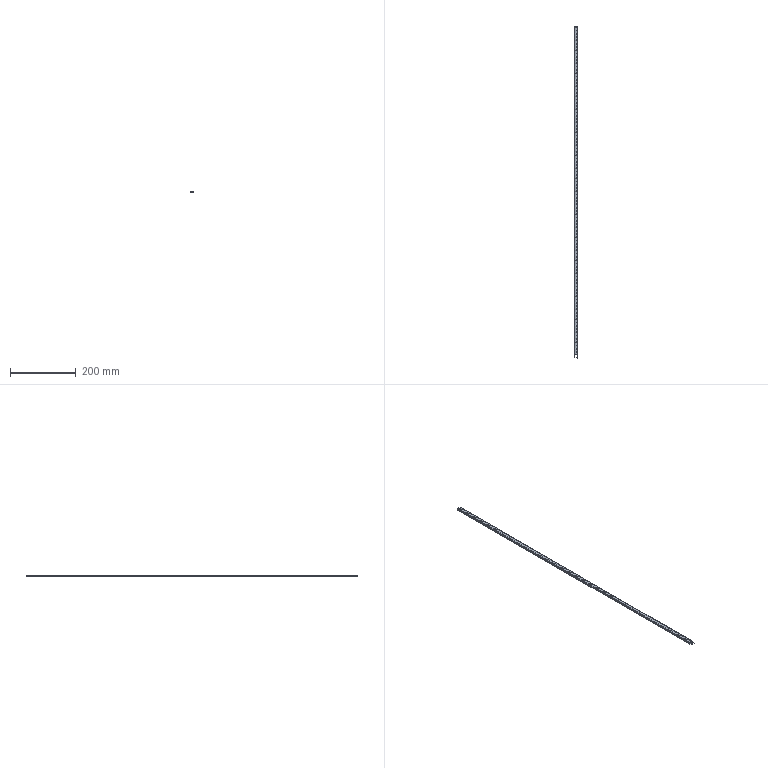Component | SolidWorks | LEDLightingStrip-2 | 1 solid | 712 faces | volume 61617 mm3 | torus 400 | cylinder 204 | plane 108 | commonest cylinder face diameters 2 x200 1.547 x2 1.337 x2